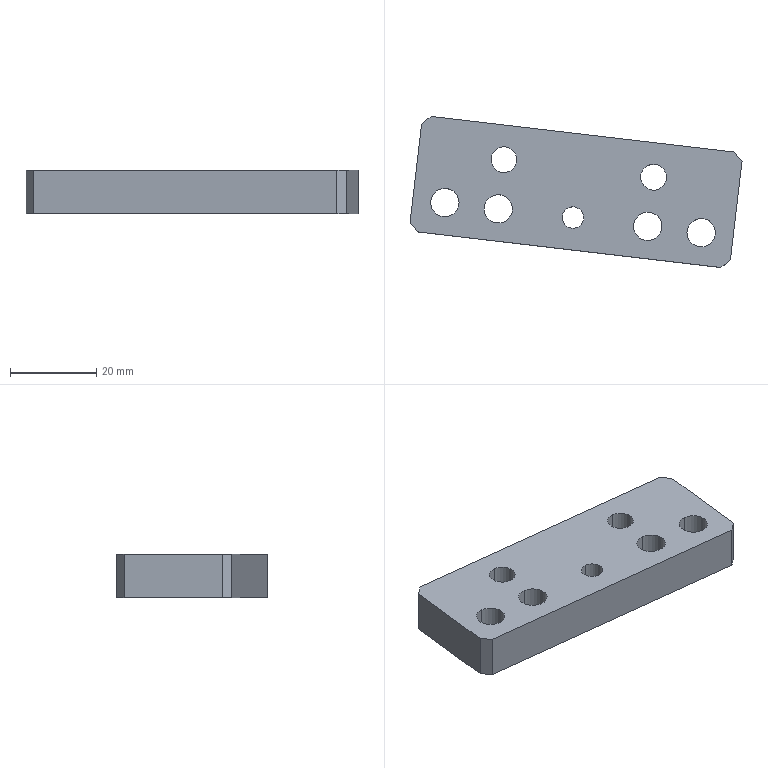Component | SolidWorks | 8TC-A17001-90-06EdgePressingRollerLockPlate-1 | 1 solid | 24 faces | box 77.17 x 35.1 x 10 mm | volume 18040 mm3 | cylinder 14 | plane 10 | commonest cylinder face diameters 6.6 x8 6 x4 5 x2 | material A3
build123d program:
from build123d import *

# Parameters (mm, degrees)
SKETCH1_W                     = 27
SKETCH1_H                     = 75
BOSS_EXTRUDE1_DEPTH           = 10
CHAMFER1_SIZE                 = 2
M6_CLEARANCE_HOLE_1_D         = 6.6
SIZE_MM_DOWEL_PIN_HOLE2_D     = 6
SIZE_MM_DOWEL_PIN_HOLE2_DEPTH = 10
SIZE_MM_DOWEL_PIN_HOLE2_TIP   = 1.803
M6_TAPPED_HOLE1_D             = 5


with BuildPart() as part:
    # Sketch1 → Boss-Extrude1 (new body)
    with BuildSketch(Plane.XY):
        Rectangle(SKETCH1_W, SKETCH1_H)
    extrude(amount=BOSS_EXTRUDE1_DEPTH)

    # Chamfer1
    chamfer1_edges = [part.edges().sort_by_distance(p)[0] for p in [
        (-13.5, 37.5, 5),
        (13.5, 37.5, 5),
        (13.5, -37.5, 5),
        (-13.5, -37.5, 5),
    ]]
    chamfer(chamfer1_edges, length=CHAMFER1_SIZE)

    # M6 Clearance Hole 1 (through all)
    with Locations(Plane.XY.offset(10)):
        with Locations((-6, 30), (-6, -30), (-6, 17.5), (-6, -17.5)):
            Hole(M6_CLEARANCE_HOLE_1_D / 2)

    # Size mm Dowel Pin Hole2
    with Locations(Plane.XY.offset(10)):
        with Locations((5.5, 17.5), (5.5, -17.5)):
            Hole(SIZE_MM_DOWEL_PIN_HOLE2_D / 2, depth=SIZE_MM_DOWEL_PIN_HOLE2_DEPTH)
            with Locations((0, 0, -(SIZE_MM_DOWEL_PIN_HOLE2_DEPTH + SIZE_MM_DOWEL_PIN_HOLE2_TIP / 2))):  # 118° drill point
                Cone(0, SIZE_MM_DOWEL_PIN_HOLE2_D / 2, SIZE_MM_DOWEL_PIN_HOLE2_TIP, mode=Mode.SUBTRACT)

    # M6 Tapped Hole1 (through all)
    with Locations(Plane.XY.offset(10)):
        with Locations((-6, 0)):
            Hole(M6_TAPPED_HOLE1_D / 2)


solid = part.part

# Placed as in the assembly
solid = solid.moved(Location((0.4951, -88.041, -136.2), (-180, 0, -83.3)))
STEP:
#1=CARTESIAN_POINT('',(-0.01955,-3.799,-5.362));
#2=VERTEX_POINT('',#1);
#3=CARTESIAN_POINT('',(0.003417,-3.603,-5.362));
#4=VERTEX_POINT('',#3);
#5=CARTESIAN_POINT('',(-0.008066,-3.701,-5.362));
#6=DIRECTION('',(-0.,0.,-1.));
#7=DIRECTION('',(0.1167,0.9932,0.));
#8=AXIS2_PLACEMENT_3D('',#5,#6,#7);
#9=CIRCLE('',#8,0.09843);
#10=EDGE_CURVE('',#2,#4,#9,.T.);
#11=ORIENTED_EDGE('',*,*,#10,.F.);
#12=CARTESIAN_POINT('',(-0.01955,-3.799,-5.756));
#13=VERTEX_POINT('',#12);
#14=CARTESIAN_POINT('',(-0.01955,-3.799,-5.756));
#15=DIRECTION('',(-0.,0.,-1.));
#16=VECTOR('',#15,39.37);
#17=LINE('',#14,#16);
#18=EDGE_CURVE('',#2,#13,#17,.T.);
#19=ORIENTED_EDGE('',*,*,#18,.T.);
#20=CARTESIAN_POINT('',(0.003417,-3.603,-5.756));
#21=VERTEX_POINT('',#20);
#22=CARTESIAN_POINT('',(-0.008066,-3.701,-5.756));
#23=DIRECTION('',(-0.,0.,-1.));
#24=DIRECTION('',(0.1167,0.9932,0.));
#25=AXIS2_PLACEMENT_3D('',#22,#23,#24);
#26=CIRCLE('',#25,0.09843);
#27=EDGE_CURVE('',#13,#21,#26,.T.);
#28=ORIENTED_EDGE('',*,*,#27,.T.);
#29=CARTESIAN_POINT('',(0.003417,-3.603,-5.756));
#30=DIRECTION('',(-0.,0.,-1.));
#31=VECTOR('',#30,39.37);
#32=LINE('',#29,#31);
#33=EDGE_CURVE('',#4,#21,#32,.T.);
#34=ORIENTED_EDGE('',*,*,#33,.F.);
#35=EDGE_LOOP('',(#11,#19,#28,#34));
#36=FACE_OUTER_BOUND('',#35,.T.);
#37=CARTESIAN_POINT('',(-0.008066,-3.701,-5.756));
#38=DIRECTION('',(-0.,0.,-1.));
#39=DIRECTION('',(0.1167,0.9932,0.));
#40=AXIS2_PLACEMENT_3D('',#37,#38,#39);
#41=CYLINDRICAL_SURFACE('',#40,0.09843);
#42=ADVANCED_FACE('',(#36),#41,.F.);
#43=CARTESIAN_POINT('',(0.7152,-3.449,-5.362));
#44=VERTEX_POINT('',#43);
#45=CARTESIAN_POINT('',(0.7428,-3.214,-5.362));
#46=VERTEX_POINT('',#45);
#47=CARTESIAN_POINT('',(0.729,-3.332,-5.362));
#48=DIRECTION('',(-0.,0.,-1.));
#49=DIRECTION('',(0.1167,0.9932,0.));
#50=AXIS2_PLACEMENT_3D('',#47,#48,#49);
#51=CIRCLE('',#50,0.1181);
#52=EDGE_CURVE('',#44,#46,#51,.T.);
#53=ORIENTED_EDGE('',*,*,#52,.F.);
#54=CARTESIAN_POINT('',(0.7152,-3.449,-5.756));
#55=VERTEX_POINT('',#54);
#56=CARTESIAN_POINT('',(0.7152,-3.449,-5.756));
#57=DIRECTION('',(-0.,0.,-1.));
#58=VECTOR('',#57,39.37);
#59=LINE('',#56,#58);
#60=EDGE_CURVE('',#44,#55,#59,.T.);
#61=ORIENTED_EDGE('',*,*,#60,.T.);
#62=CARTESIAN_POINT('',(0.7428,-3.214,-5.756));
#63=VERTEX_POINT('',#62);
#64=CARTESIAN_POINT('',(0.729,-3.332,-5.756));
#65=DIRECTION('',(-0.,0.,-1.));
#66=DIRECTION('',(0.1167,0.9932,0.));
#67=AXIS2_PLACEMENT_3D('',#64,#65,#66);
#68=CIRCLE('',#67,0.1181);
#69=EDGE_CURVE('',#55,#63,#68,.T.);
#70=ORIENTED_EDGE('',*,*,#69,.T.);
#71=CARTESIAN_POINT('',(0.7428,-3.214,-5.756));
#72=DIRECTION('',(-0.,0.,-1.));
#73=VECTOR('',#72,39.37);
#74=LINE('',#71,#73);
#75=EDGE_CURVE('',#46,#63,#74,.T.);
#76=ORIENTED_EDGE('',*,*,#75,.F.);
#77=EDGE_LOOP('',(#53,#61,#70,#76));
#78=FACE_OUTER_BOUND('',#77,.T.);
#79=CARTESIAN_POINT('',(0.729,-3.332,-5.756));
#80=DIRECTION('',(-0.,0.,-1.));
#81=DIRECTION('',(0.1167,0.9932,0.));
#82=AXIS2_PLACEMENT_3D('',#79,#80,#81);
#83=CYLINDRICAL_SURFACE('',#82,0.1181);
#84=ADVANCED_FACE('',(#78),#83,.F.);
#85=CARTESIAN_POINT('',(-0.6533,-3.288,-5.362));
#86=VERTEX_POINT('',#85);
#87=CARTESIAN_POINT('',(-0.6257,-3.053,-5.362));
#88=VERTEX_POINT('',#87);
#89=CARTESIAN_POINT('',(-0.6395,-3.171,-5.362));
#90=DIRECTION('',(-0.,0.,-1.));
#91=DIRECTION('',(0.1167,0.9932,0.));
#92=AXIS2_PLACEMENT_3D('',#89,#90,#91);
#93=CIRCLE('',#92,0.1181);
#94=EDGE_CURVE('',#86,#88,#93,.T.);
#95=ORIENTED_EDGE('',*,*,#94,.F.);
#96=CARTESIAN_POINT('',(-0.6533,-3.288,-5.756));
#97=VERTEX_POINT('',#96);
#98=CARTESIAN_POINT('',(-0.6533,-3.288,-5.756));
#99=DIRECTION('',(-0.,0.,-1.));
#100=VECTOR('',#99,39.37);
#101=LINE('',#98,#100);
#102=EDGE_CURVE('',#86,#97,#101,.T.);
#103=ORIENTED_EDGE('',*,*,#102,.T.);
#104=CARTESIAN_POINT('',(-0.6257,-3.053,-5.756));
#105=VERTEX_POINT('',#104);
#106=CARTESIAN_POINT('',(-0.6395,-3.171,-5.756));
#107=DIRECTION('',(-0.,0.,-1.));
#108=DIRECTION('',(0.1167,0.9932,0.));
#109=AXIS2_PLACEMENT_3D('',#106,#107,#108);
#110=CIRCLE('',#109,0.1181);
#111=EDGE_CURVE('',#97,#105,#110,.T.);
#112=ORIENTED_EDGE('',*,*,#111,.T.);
#113=CARTESIAN_POINT('',(-0.6257,-3.053,-5.756));
#114=DIRECTION('',(-0.,0.,-1.));
#115=VECTOR('',#114,39.37);
#116=LINE('',#113,#115);
#117=EDGE_CURVE('',#88,#105,#116,.T.);
#118=ORIENTED_EDGE('',*,*,#117,.F.);
#119=EDGE_LOOP('',(#95,#103,#112,#118));
#120=FACE_OUTER_BOUND('',#119,.T.);
#121=CARTESIAN_POINT('',(-0.6395,-3.171,-5.756));
#122=DIRECTION('',(-0.,0.,-1.));
#123=DIRECTION('',(0.1167,0.9932,0.));
#124=AXIS2_PLACEMENT_3D('',#121,#122,#123);
#125=CYLINDRICAL_SURFACE('',#124,0.1181);
#126=ADVANCED_FACE('',(#120),#125,.F.);
#127=CARTESIAN_POINT('',(1.15,-3.968,-5.362));
#128=VERTEX_POINT('',#127);
#129=CARTESIAN_POINT('',(1.18,-3.71,-5.362));
#130=VERTEX_POINT('',#129);
#131=CARTESIAN_POINT('',(1.165,-3.839,-5.362));
#132=DIRECTION('',(-0.,0.,-1.));
#133=DIRECTION('',(0.1167,0.9932,0.));
#134=AXIS2_PLACEMENT_3D('',#131,#132,#133);
#135=CIRCLE('',#134,0.1299);
#136=EDGE_CURVE('',#128,#130,#135,.T.);
#137=ORIENTED_EDGE('',*,*,#136,.F.);
#138=CARTESIAN_POINT('',(1.15,-3.968,-5.756));
#139=VERTEX_POINT('',#138);
#140=CARTESIAN_POINT('',(1.15,-3.968,-5.756));
#141=DIRECTION('',(-0.,0.,-1.));
#142=VECTOR('',#141,39.37);
#143=LINE('',#140,#142);
#144=EDGE_CURVE('',#128,#139,#143,.T.);
#145=ORIENTED_EDGE('',*,*,#144,.T.);
#146=CARTESIAN_POINT('',(1.18,-3.71,-5.756));
#147=VERTEX_POINT('',#146);
#148=CARTESIAN_POINT('',(1.165,-3.839,-5.756));
#149=DIRECTION('',(-0.,0.,-1.));
#150=DIRECTION('',(0.1167,0.9932,0.));
#151=AXIS2_PLACEMENT_3D('',#148,#149,#150);
#152=CIRCLE('',#151,0.1299);
#153=EDGE_CURVE('',#139,#147,#152,.T.);
#154=ORIENTED_EDGE('',*,*,#153,.T.);
#155=CARTESIAN_POINT('',(1.18,-3.71,-5.756));
#156=DIRECTION('',(-0.,0.,-1.));
#157=VECTOR('',#156,39.37);
#158=LINE('',#155,#157);
#159=EDGE_CURVE('',#130,#147,#158,.T.);
#160=ORIENTED_EDGE('',*,*,#159,.F.);
#161=EDGE_LOOP('',(#137,#145,#154,#160));
#162=FACE_OUTER_BOUND('',#161,.T.);
#163=CARTESIAN_POINT('',(1.165,-3.839,-5.756));
#164=DIRECTION('',(-0.,0.,-1.));
#165=DIRECTION('',(0.1167,0.9932,0.));
#166=AXIS2_PLACEMENT_3D('',#163,#164,#165);
#167=CYLINDRICAL_SURFACE('',#166,0.1299);
#168=ADVANCED_FACE('',(#162),#167,.F.);
#169=CARTESIAN_POINT('',(-1.196,-3.692,-5.362));
#170=VERTEX_POINT('',#169);
#171=CARTESIAN_POINT('',(-1.166,-3.434,-5.362));
#172=VERTEX_POINT('',#171);
#173=CARTESIAN_POINT('',(-1.181,-3.563,-5.362));
#174=DIRECTION('',(-0.,0.,-1.));
#175=DIRECTION('',(0.1167,0.9932,0.));
#176=AXIS2_PLACEMENT_3D('',#173,#174,#175);
#177=CIRCLE('',#176,0.1299);
#178=EDGE_CURVE('',#170,#172,#177,.T.);
#179=ORIENTED_EDGE('',*,*,#178,.F.);
#180=CARTESIAN_POINT('',(-1.196,-3.692,-5.756));
#181=VERTEX_POINT('',#180);
#182=CARTESIAN_POINT('',(-1.196,-3.692,-5.756));
#183=DIRECTION('',(-0.,0.,-1.));
#184=VECTOR('',#183,39.37);
#185=LINE('',#182,#184);
#186=EDGE_CURVE('',#170,#181,#185,.T.);
#187=ORIENTED_EDGE('',*,*,#186,.T.);
#188=CARTESIAN_POINT('',(-1.166,-3.434,-5.756));
#189=VERTEX_POINT('',#188);
#190=CARTESIAN_POINT('',(-1.181,-3.563,-5.756));
#191=DIRECTION('',(-0.,0.,-1.));
#192=DIRECTION('',(0.1167,0.9932,0.));
#193=AXIS2_PLACEMENT_3D('',#190,#191,#192);
#194=CIRCLE('',#193,0.1299);
#195=EDGE_CURVE('',#181,#189,#194,.T.);
#196=ORIENTED_EDGE('',*,*,#195,.T.);
#197=CARTESIAN_POINT('',(-1.166,-3.434,-5.756));
#198=DIRECTION('',(-0.,0.,-1.));
#199=VECTOR('',#198,39.37);
#200=LINE('',#197,#199);
#201=EDGE_CURVE('',#172,#189,#200,.T.);
#202=ORIENTED_EDGE('',*,*,#201,.F.);
#203=EDGE_LOOP('',(#179,#187,#196,#202));
#204=FACE_OUTER_BOUND('',#203,.T.);
#205=CARTESIAN_POINT('',(-1.181,-3.563,-5.756));
#206=DIRECTION('',(-0.,0.,-1.));
#207=DIRECTION('',(0.1167,0.9932,0.));
#208=AXIS2_PLACEMENT_3D('',#205,#206,#207);
#209=CYLINDRICAL_SURFACE('',#208,0.1299);
#210=ADVANCED_FACE('',(#204),#209,.F.);
#211=CARTESIAN_POINT('',(0.661,-3.91,-5.362));
#212=VERTEX_POINT('',#211);
#213=CARTESIAN_POINT('',(0.6914,-3.652,-5.362));
#214=VERTEX_POINT('',#213);
#215=CARTESIAN_POINT('',(0.6762,-3.781,-5.362));
#216=DIRECTION('',(-0.,0.,-1.));
#217=DIRECTION('',(0.1167,0.9932,0.));
#218=AXIS2_PLACEMENT_3D('',#215,#216,#217);
#219=CIRCLE('',#218,0.1299);
#220=EDGE_CURVE('',#212,#214,#219,.T.);
#221=ORIENTED_EDGE('',*,*,#220,.F.);
#222=CARTESIAN_POINT('',(0.661,-3.91,-5.756));
#223=VERTEX_POINT('',#222);
#224=CARTESIAN_POINT('',(0.661,-3.91,-5.756));
#225=DIRECTION('',(-0.,0.,-1.));
#226=VECTOR('',#225,39.37);
#227=LINE('',#224,#226);
#228=EDGE_CURVE('',#212,#223,#227,.T.);
#229=ORIENTED_EDGE('',*,*,#228,.T.);
#230=CARTESIAN_POINT('',(0.6914,-3.652,-5.756));
#231=VERTEX_POINT('',#230);
#232=CARTESIAN_POINT('',(0.6762,-3.781,-5.756));
#233=DIRECTION('',(-0.,0.,-1.));
#234=DIRECTION('',(0.1167,0.9932,0.));
#235=AXIS2_PLACEMENT_3D('',#232,#233,#234);
#236=CIRCLE('',#235,0.1299);
#237=EDGE_CURVE('',#223,#231,#236,.T.);
#238=ORIENTED_EDGE('',*,*,#237,.T.);
#239=CARTESIAN_POINT('',(0.6914,-3.652,-5.756));
#240=DIRECTION('',(-0.,0.,-1.));
#241=VECTOR('',#240,39.37);
#242=LINE('',#239,#241);
#243=EDGE_CURVE('',#214,#231,#242,.T.);
#244=ORIENTED_EDGE('',*,*,#243,.F.);
#245=EDGE_LOOP('',(#221,#229,#238,#244));
#246=FACE_OUTER_BOUND('',#245,.T.);
#247=CARTESIAN_POINT('',(0.6762,-3.781,-5.756));
#248=DIRECTION('',(-0.,0.,-1.));
#249=DIRECTION('',(0.1167,0.9932,0.));
#250=AXIS2_PLACEMENT_3D('',#247,#248,#249);
#251=CYLINDRICAL_SURFACE('',#250,0.1299);
#252=ADVANCED_FACE('',(#246),#251,.F.);
#253=CARTESIAN_POINT('',(-0.7075,-3.749,-5.362));
#254=VERTEX_POINT('',#253);
#255=CARTESIAN_POINT('',(-0.6772,-3.491,-5.362));
#256=VERTEX_POINT('',#255);
#257=CARTESIAN_POINT('',(-0.6923,-3.62,-5.362));
#258=DIRECTION('',(-0.,0.,-1.));
#259=DIRECTION('',(0.1167,0.9932,0.));
#260=AXIS2_PLACEMENT_3D('',#257,#258,#259);
#261=CIRCLE('',#260,0.1299);
#262=EDGE_CURVE('',#254,#256,#261,.T.);
#263=ORIENTED_EDGE('',*,*,#262,.F.);
#264=CARTESIAN_POINT('',(-0.7075,-3.749,-5.756));
#265=VERTEX_POINT('',#264);
#266=CARTESIAN_POINT('',(-0.7075,-3.749,-5.756));
#267=DIRECTION('',(-0.,0.,-1.));
#268=VECTOR('',#267,39.37);
#269=LINE('',#266,#268);
#270=EDGE_CURVE('',#254,#265,#269,.T.);
#271=ORIENTED_EDGE('',*,*,#270,.T.);
#272=CARTESIAN_POINT('',(-0.6772,-3.491,-5.756));
#273=VERTEX_POINT('',#272);
#274=CARTESIAN_POINT('',(-0.6923,-3.62,-5.756));
#275=DIRECTION('',(-0.,0.,-1.));
#276=DIRECTION('',(0.1167,0.9932,0.));
#277=AXIS2_PLACEMENT_3D('',#274,#275,#276);
#278=CIRCLE('',#277,0.1299);
#279=EDGE_CURVE('',#265,#273,#278,.T.);
#280=ORIENTED_EDGE('',*,*,#279,.T.);
#281=CARTESIAN_POINT('',(-0.6772,-3.491,-5.756));
#282=DIRECTION('',(-0.,0.,-1.));
#283=VECTOR('',#282,39.37);
#284=LINE('',#281,#283);
#285=EDGE_CURVE('',#256,#273,#284,.T.);
#286=ORIENTED_EDGE('',*,*,#285,.F.);
#287=EDGE_LOOP('',(#263,#271,#280,#286));
#288=FACE_OUTER_BOUND('',#287,.T.);
#289=CARTESIAN_POINT('',(-0.6923,-3.62,-5.756));
#290=DIRECTION('',(-0.,0.,-1.));
#291=DIRECTION('',(0.1167,0.9932,0.));
#292=AXIS2_PLACEMENT_3D('',#289,#290,#291);
#293=CYLINDRICAL_SURFACE('',#292,0.1299);
#294=ADVANCED_FACE('',(#288),#293,.F.);
#295=CARTESIAN_POINT('',(1.346,-4.157,-5.362));
#296=VERTEX_POINT('',#295);
#297=CARTESIAN_POINT('',(-1.431,-3.831,-5.362));
#298=VERTEX_POINT('',#297);
#299=CARTESIAN_POINT('',(1.424,-4.166,-5.362));
#300=DIRECTION('',(-0.9932,0.1167,0.));
#301=VECTOR('',#300,39.37);
#302=LINE('',#299,#301);
#303=EDGE_CURVE('',#296,#298,#302,.T.);
#304=ORIENTED_EDGE('',*,*,#303,.T.);
#305=CARTESIAN_POINT('',(-1.431,-3.831,-5.756));
#306=VERTEX_POINT('',#305);
#307=CARTESIAN_POINT('',(-1.431,-3.831,-5.756));
#308=DIRECTION('',(-0.,0.,-1.));
#309=VECTOR('',#308,39.37);
#310=LINE('',#307,#309);
#311=EDGE_CURVE('',#298,#306,#310,.T.);
#312=ORIENTED_EDGE('',*,*,#311,.T.);
#313=CARTESIAN_POINT('',(1.346,-4.157,-5.756));
#314=VERTEX_POINT('',#313);
#315=CARTESIAN_POINT('',(1.424,-4.166,-5.756));
#316=DIRECTION('',(-0.9932,0.1167,0.));
#317=VECTOR('',#316,39.37);
#318=LINE('',#315,#317);
#319=EDGE_CURVE('',#314,#306,#318,.T.);
#320=ORIENTED_EDGE('',*,*,#319,.F.);
#321=CARTESIAN_POINT('',(1.346,-4.157,-5.756));
#322=DIRECTION('',(0.,-0.,1.));
#323=VECTOR('',#322,39.37);
#324=LINE('',#321,#323);
#325=EDGE_CURVE('',#314,#296,#324,.T.);
#326=ORIENTED_EDGE('',*,*,#325,.T.);
#327=EDGE_LOOP('',(#304,#312,#320,#326));
#328=FACE_OUTER_BOUND('',#327,.T.);
#329=CARTESIAN_POINT('',(1.424,-4.166,-5.756));
#330=DIRECTION('',(0.1167,0.9932,0.));
#331=DIRECTION('',(0.9932,-0.1167,-0.));
#332=AXIS2_PLACEMENT_3D('',#329,#330,#331);
#333=PLANE('',#332);
#334=ADVANCED_FACE('',(#328),#333,.F.);
#335=CARTESIAN_POINT('',(-1.5,-3.744,-5.756));
#336=VERTEX_POINT('',#335);
#337=CARTESIAN_POINT('',(-1.394,-2.844,-5.756));
#338=VERTEX_POINT('',#337);
#339=CARTESIAN_POINT('',(-1.385,-2.766,-5.756));
#340=DIRECTION('',(0.1167,0.9932,0.));
#341=VECTOR('',#340,39.37);
#342=LINE('',#339,#341);
#343=EDGE_CURVE('',#336,#338,#342,.T.);
#344=ORIENTED_EDGE('',*,*,#343,.F.);
#345=CARTESIAN_POINT('',(-1.5,-3.744,-5.362));
#346=VERTEX_POINT('',#345);
#347=CARTESIAN_POINT('',(-1.5,-3.744,-5.756));
#348=DIRECTION('',(0.,-0.,1.));
#349=VECTOR('',#348,39.37);
#350=LINE('',#347,#349);
#351=EDGE_CURVE('',#336,#346,#350,.T.);
#352=ORIENTED_EDGE('',*,*,#351,.T.);
#353=CARTESIAN_POINT('',(-1.394,-2.844,-5.362));
#354=VERTEX_POINT('',#353);
#355=CARTESIAN_POINT('',(-1.385,-2.766,-5.362));
#356=DIRECTION('',(0.1167,0.9932,0.));
#357=VECTOR('',#356,39.37);
#358=LINE('',#355,#357);
#359=EDGE_CURVE('',#346,#354,#358,.T.);
#360=ORIENTED_EDGE('',*,*,#359,.T.);
#361=CARTESIAN_POINT('',(-1.394,-2.844,-5.756));
#362=DIRECTION('',(-0.,0.,-1.));
#363=VECTOR('',#362,39.37);
#364=LINE('',#361,#363);
#365=EDGE_CURVE('',#354,#338,#364,.T.);
#366=ORIENTED_EDGE('',*,*,#365,.T.);
#367=EDGE_LOOP('',(#344,#352,#360,#366));
#368=FACE_OUTER_BOUND('',#367,.T.);
#369=CARTESIAN_POINT('',(-1.385,-2.766,-5.756));
#370=DIRECTION('',(0.9932,-0.1167,-0.));
#371=DIRECTION('',(-0.,0.,-1.));
#372=AXIS2_PLACEMENT_3D('',#369,#370,#371);
#373=PLANE('',#372);
#374=ADVANCED_FACE('',(#368),#373,.F.);
#375=CARTESIAN_POINT('',(-1.307,-2.775,-5.756));
#376=VERTEX_POINT('',#375);
#377=CARTESIAN_POINT('',(1.47,-3.101,-5.756));
#378=VERTEX_POINT('',#377);
#379=CARTESIAN_POINT('',(1.548,-3.111,-5.756));
#380=DIRECTION('',(0.9932,-0.1167,-0.));
#381=VECTOR('',#380,39.37);
#382=LINE('',#379,#381);
#383=EDGE_CURVE('',#376,#378,#382,.T.);
#384=ORIENTED_EDGE('',*,*,#383,.F.);
#385=CARTESIAN_POINT('',(-1.307,-2.775,-5.362));
#386=VERTEX_POINT('',#385);
#387=CARTESIAN_POINT('',(-1.307,-2.775,-5.756));
#388=DIRECTION('',(0.,-0.,1.));
#389=VECTOR('',#388,39.37);
#390=LINE('',#387,#389);
#391=EDGE_CURVE('',#376,#386,#390,.T.);
#392=ORIENTED_EDGE('',*,*,#391,.T.);
#393=CARTESIAN_POINT('',(1.47,-3.101,-5.362));
#394=VERTEX_POINT('',#393);
#395=CARTESIAN_POINT('',(1.548,-3.111,-5.362));
#396=DIRECTION('',(0.9932,-0.1167,-0.));
#397=VECTOR('',#396,39.37);
#398=LINE('',#395,#397);
#399=EDGE_CURVE('',#386,#394,#398,.T.);
#400=ORIENTED_EDGE('',*,*,#399,.T.);
#401=CARTESIAN_POINT('',(1.47,-3.101,-5.756));
#402=DIRECTION('',(-0.,0.,-1.));
#403=VECTOR('',#402,39.37);
#404=LINE('',#401,#403);
#405=EDGE_CURVE('',#394,#378,#404,.T.);
#406=ORIENTED_EDGE('',*,*,#405,.T.);
#407=EDGE_LOOP('',(#384,#392,#400,#406));
#408=FACE_OUTER_BOUND('',#407,.T.);
#409=CARTESIAN_POINT('',(1.548,-3.111,-5.756));
#410=DIRECTION('',(-0.1167,-0.9932,-0.));
#411=DIRECTION('',(-0.9932,0.1167,0.));
#412=AXIS2_PLACEMENT_3D('',#409,#410,#411);
#413=PLANE('',#412);
#414=ADVANCED_FACE('',(#408),#413,.F.);
#415=CARTESIAN_POINT('',(1.539,-3.189,-5.362));
#416=VERTEX_POINT('',#415);
#417=CARTESIAN_POINT('',(1.433,-4.088,-5.362));
#418=VERTEX_POINT('',#417);
#419=CARTESIAN_POINT('',(1.548,-3.111,-5.362));
#420=DIRECTION('',(-0.1167,-0.9932,-0.));
#421=VECTOR('',#420,39.37);
#422=LINE('',#419,#421);
#423=EDGE_CURVE('',#416,#418,#422,.T.);
#424=ORIENTED_EDGE('',*,*,#423,.T.);
#425=CARTESIAN_POINT('',(1.433,-4.088,-5.756));
#426=VERTEX_POINT('',#425);
#427=CARTESIAN_POINT('',(1.433,-4.088,-5.756));
#428=DIRECTION('',(-0.,0.,-1.));
#429=VECTOR('',#428,39.37);
#430=LINE('',#427,#429);
#431=EDGE_CURVE('',#418,#426,#430,.T.);
#432=ORIENTED_EDGE('',*,*,#431,.T.);
#433=CARTESIAN_POINT('',(1.539,-3.189,-5.756));
#434=VERTEX_POINT('',#433);
#435=CARTESIAN_POINT('',(1.548,-3.111,-5.756));
#436=DIRECTION('',(-0.1167,-0.9932,-0.));
#437=VECTOR('',#436,39.37);
#438=LINE('',#435,#437);
#439=EDGE_CURVE('',#434,#426,#438,.T.);
#440=ORIENTED_EDGE('',*,*,#439,.F.);
#441=CARTESIAN_POINT('',(1.539,-3.189,-5.756));
#442=DIRECTION('',(0.,-0.,1.));
#443=VECTOR('',#442,39.37);
#444=LINE('',#441,#443);
#445=EDGE_CURVE('',#434,#416,#444,.T.);
#446=ORIENTED_EDGE('',*,*,#445,.T.);
#447=EDGE_LOOP('',(#424,#432,#440,#446));
#448=FACE_OUTER_BOUND('',#447,.T.);
#449=CARTESIAN_POINT('',(1.548,-3.111,-5.756));
#450=DIRECTION('',(-0.9932,0.1167,0.));
#451=DIRECTION('',(0.,-0.,1.));
#452=AXIS2_PLACEMENT_3D('',#449,#450,#451);
#453=PLANE('',#452);
#454=ADVANCED_FACE('',(#448),#453,.F.);
#455=CARTESIAN_POINT('',(-0.008066,-3.701,-5.756));
#456=DIRECTION('',(-0.,0.,-1.));
#457=DIRECTION('',(0.1167,0.9932,0.));
#458=AXIS2_PLACEMENT_3D('',#455,#456,#457);
#459=CIRCLE('',#458,0.09843);
#460=EDGE_CURVE('',#21,#13,#459,.T.);
#461=ORIENTED_EDGE('',*,*,#460,.F.);
#462=ORIENTED_EDGE('',*,*,#27,.F.);
#463=EDGE_LOOP('',(#461,#462));
#464=FACE_BOUND('',#463,.T.);
#465=CARTESIAN_POINT('',(0.729,-3.332,-5.756));
#466=DIRECTION('',(-0.,0.,-1.));
#467=DIRECTION('',(0.1167,0.9932,0.));
#468=AXIS2_PLACEMENT_3D('',#465,#466,#467);
#469=CIRCLE('',#468,0.1181);
#470=EDGE_CURVE('',#63,#55,#469,.T.);
#471=ORIENTED_EDGE('',*,*,#470,.F.);
#472=ORIENTED_EDGE('',*,*,#69,.F.);
#473=EDGE_LOOP('',(#471,#472));
#474=FACE_BOUND('',#473,.T.);
#475=CARTESIAN_POINT('',(-0.6395,-3.171,-5.756));
#476=DIRECTION('',(-0.,0.,-1.));
#477=DIRECTION('',(0.1167,0.9932,0.));
#478=AXIS2_PLACEMENT_3D('',#475,#476,#477);
#479=CIRCLE('',#478,0.1181);
#480=EDGE_CURVE('',#105,#97,#479,.T.);
#481=ORIENTED_EDGE('',*,*,#480,.F.);
#482=ORIENTED_EDGE('',*,*,#111,.F.);
#483=EDGE_LOOP('',(#481,#482));
#484=FACE_BOUND('',#483,.T.);
#485=CARTESIAN_POINT('',(1.165,-3.839,-5.756));
#486=DIRECTION('',(-0.,0.,-1.));
#487=DIRECTION('',(0.1167,0.9932,0.));
#488=AXIS2_PLACEMENT_3D('',#485,#486,#487);
#489=CIRCLE('',#488,0.1299);
#490=EDGE_CURVE('',#147,#139,#489,.T.);
#491=ORIENTED_EDGE('',*,*,#490,.F.);
#492=ORIENTED_EDGE('',*,*,#153,.F.);
#493=EDGE_LOOP('',(#491,#492));
#494=FACE_BOUND('',#493,.T.);
#495=CARTESIAN_POINT('',(-1.181,-3.563,-5.756));
#496=DIRECTION('',(-0.,0.,-1.));
#497=DIRECTION('',(0.1167,0.9932,0.));
#498=AXIS2_PLACEMENT_3D('',#495,#496,#497);
#499=CIRCLE('',#498,0.1299);
#500=EDGE_CURVE('',#189,#181,#499,.T.);
#501=ORIENTED_EDGE('',*,*,#500,.F.);
#502=ORIENTED_EDGE('',*,*,#195,.F.);
#503=EDGE_LOOP('',(#501,#502));
#504=FACE_BOUND('',#503,.T.);
#505=CARTESIAN_POINT('',(0.6762,-3.781,-5.756));
#506=DIRECTION('',(-0.,0.,-1.));
#507=DIRECTION('',(0.1167,0.9932,0.));
#508=AXIS2_PLACEMENT_3D('',#505,#506,#507);
#509=CIRCLE('',#508,0.1299);
#510=EDGE_CURVE('',#231,#223,#509,.T.);
#511=ORIENTED_EDGE('',*,*,#510,.F.);
#512=ORIENTED_EDGE('',*,*,#237,.F.);
#513=EDGE_LOOP('',(#511,#512));
#514=FACE_BOUND('',#513,.T.);
#515=CARTESIAN_POINT('',(-0.6923,-3.62,-5.756));
#516=DIRECTION('',(-0.,0.,-1.));
#517=DIRECTION('',(0.1167,0.9932,0.));
#518=AXIS2_PLACEMENT_3D('',#515,#516,#517);
#519=CIRCLE('',#518,0.1299);
#520=EDGE_CURVE('',#273,#265,#519,.T.);
#521=ORIENTED_EDGE('',*,*,#520,.F.);
#522=ORIENTED_EDGE('',*,*,#279,.F.);
#523=EDGE_LOOP('',(#521,#522));
#524=FACE_BOUND('',#523,.T.);
#525=ORIENTED_EDGE('',*,*,#319,.T.);
#526=CARTESIAN_POINT('',(-1.5,-3.744,-5.756));
#527=DIRECTION('',(-0.6198,0.7848,0.));
#528=VECTOR('',#527,39.37);
#529=LINE('',#526,#528);
#530=EDGE_CURVE('',#306,#336,#529,.T.);
#531=ORIENTED_EDGE('',*,*,#530,.T.);
#532=ORIENTED_EDGE('',*,*,#343,.T.);
#533=CARTESIAN_POINT('',(-1.307,-2.775,-5.756));
#534=DIRECTION('',(0.7848,0.6198,0.));
#535=VECTOR('',#534,39.37);
#536=LINE('',#533,#535);
#537=EDGE_CURVE('',#338,#376,#536,.T.);
#538=ORIENTED_EDGE('',*,*,#537,.T.);
#539=ORIENTED_EDGE('',*,*,#383,.T.);
#540=CARTESIAN_POINT('',(1.539,-3.189,-5.756));
#541=DIRECTION('',(0.6198,-0.7848,-0.));
#542=VECTOR('',#541,39.37);
#543=LINE('',#540,#542);
#544=EDGE_CURVE('',#378,#434,#543,.T.);
#545=ORIENTED_EDGE('',*,*,#544,.T.);
#546=ORIENTED_EDGE('',*,*,#439,.T.);
#547=CARTESIAN_POINT('',(1.346,-4.157,-5.756));
#548=DIRECTION('',(-0.7848,-0.6198,-0.));
#549=VECTOR('',#548,39.37);
#550=LINE('',#547,#549);
#551=EDGE_CURVE('',#426,#314,#550,.T.);
#552=ORIENTED_EDGE('',*,*,#551,.T.);
#553=EDGE_LOOP('',(#525,#531,#532,#538,#539,#545,#546,#552));
#554=FACE_OUTER_BOUND('',#553,.T.);
#555=CARTESIAN_POINT('',(0.01949,-3.466,-5.756));
#556=DIRECTION('',(0.,-0.,1.));
#557=DIRECTION('',(-0.1167,-0.9932,-0.));
#558=AXIS2_PLACEMENT_3D('',#555,#556,#557);
#559=PLANE('',#558);
#560=ADVANCED_FACE('',(#464,#474,#484,#494,#504,#514,#524,#554),#559,.F.);
#561=CARTESIAN_POINT('',(-0.008066,-3.701,-5.362));
#562=DIRECTION('',(-0.,0.,-1.));
#563=DIRECTION('',(0.1167,0.9932,0.));
#564=AXIS2_PLACEMENT_3D('',#561,#562,#563);
#565=CIRCLE('',#564,0.09843);
#566=EDGE_CURVE('',#4,#2,#565,.T.);
#567=ORIENTED_EDGE('',*,*,#566,.T.);
#568=ORIENTED_EDGE('',*,*,#10,.T.);
#569=EDGE_LOOP('',(#567,#568));
#570=FACE_BOUND('',#569,.T.);
#571=CARTESIAN_POINT('',(0.729,-3.332,-5.362));
#572=DIRECTION('',(-0.,0.,-1.));
#573=DIRECTION('',(0.1167,0.9932,0.));
#574=AXIS2_PLACEMENT_3D('',#571,#572,#573);
#575=CIRCLE('',#574,0.1181);
#576=EDGE_CURVE('',#46,#44,#575,.T.);
#577=ORIENTED_EDGE('',*,*,#576,.T.);
#578=ORIENTED_EDGE('',*,*,#52,.T.);
#579=EDGE_LOOP('',(#577,#578));
#580=FACE_BOUND('',#579,.T.);
#581=CARTESIAN_POINT('',(-0.6395,-3.171,-5.362));
#582=DIRECTION('',(-0.,0.,-1.));
#583=DIRECTION('',(0.1167,0.9932,0.));
#584=AXIS2_PLACEMENT_3D('',#581,#582,#583);
#585=CIRCLE('',#584,0.1181);
#586=EDGE_CURVE('',#88,#86,#585,.T.);
#587=ORIENTED_EDGE('',*,*,#586,.T.);
#588=ORIENTED_EDGE('',*,*,#94,.T.);
#589=EDGE_LOOP('',(#587,#588));
#590=FACE_BOUND('',#589,.T.);
#591=CARTESIAN_POINT('',(1.165,-3.839,-5.362));
#592=DIRECTION('',(-0.,0.,-1.));
#593=DIRECTION('',(0.1167,0.9932,0.));
#594=AXIS2_PLACEMENT_3D('',#591,#592,#593);
#595=CIRCLE('',#594,0.1299);
#596=EDGE_CURVE('',#130,#128,#595,.T.);
#597=ORIENTED_EDGE('',*,*,#596,.T.);
#598=ORIENTED_EDGE('',*,*,#136,.T.);
#599=EDGE_LOOP('',(#597,#598));
#600=FACE_BOUND('',#599,.T.);
#601=CARTESIAN_POINT('',(-1.181,-3.563,-5.362));
#602=DIRECTION('',(-0.,0.,-1.));
#603=DIRECTION('',(0.1167,0.9932,0.));
#604=AXIS2_PLACEMENT_3D('',#601,#602,#603);
#605=CIRCLE('',#604,0.1299);
#606=EDGE_CURVE('',#172,#170,#605,.T.);
#607=ORIENTED_EDGE('',*,*,#606,.T.);
#608=ORIENTED_EDGE('',*,*,#178,.T.);
#609=EDGE_LOOP('',(#607,#608));
#610=FACE_BOUND('',#609,.T.);
#611=CARTESIAN_POINT('',(0.6762,-3.781,-5.362));
#612=DIRECTION('',(-0.,0.,-1.));
#613=DIRECTION('',(0.1167,0.9932,0.));
#614=AXIS2_PLACEMENT_3D('',#611,#612,#613);
#615=CIRCLE('',#614,0.1299);
#616=EDGE_CURVE('',#214,#212,#615,.T.);
#617=ORIENTED_EDGE('',*,*,#616,.T.);
#618=ORIENTED_EDGE('',*,*,#220,.T.);
#619=EDGE_LOOP('',(#617,#618));
#620=FACE_BOUND('',#619,.T.);
#621=CARTESIAN_POINT('',(-0.6923,-3.62,-5.362));
#622=DIRECTION('',(-0.,0.,-1.));
#623=DIRECTION('',(0.1167,0.9932,0.));
#624=AXIS2_PLACEMENT_3D('',#621,#622,#623);
#625=CIRCLE('',#624,0.1299);
#626=EDGE_CURVE('',#256,#254,#625,.T.);
#627=ORIENTED_EDGE('',*,*,#626,.T.);
#628=ORIENTED_EDGE('',*,*,#262,.T.);
#629=EDGE_LOOP('',(#627,#628));
#630=FACE_BOUND('',#629,.T.);
#631=ORIENTED_EDGE('',*,*,#359,.F.);
#632=CARTESIAN_POINT('',(-1.051,-4.312,-5.362));
#633=DIRECTION('',(0.6198,-0.7848,-0.));
#634=VECTOR('',#633,39.37);
#635=LINE('',#632,#634);
#636=EDGE_CURVE('',#346,#298,#635,.T.);
#637=ORIENTED_EDGE('',*,*,#636,.T.);
#638=ORIENTED_EDGE('',*,*,#303,.F.);
#639=CARTESIAN_POINT('',(0.8649,-4.537,-5.362));
#640=DIRECTION('',(0.7848,0.6198,0.));
#641=VECTOR('',#640,39.37);
#642=LINE('',#639,#641);
#643=EDGE_CURVE('',#296,#418,#642,.T.);
#644=ORIENTED_EDGE('',*,*,#643,.T.);
#645=ORIENTED_EDGE('',*,*,#423,.F.);
#646=CARTESIAN_POINT('',(1.09,-2.621,-5.362));
#647=DIRECTION('',(-0.6198,0.7848,0.));
#648=VECTOR('',#647,39.37);
#649=LINE('',#646,#648);
#650=EDGE_CURVE('',#416,#394,#649,.T.);
#651=ORIENTED_EDGE('',*,*,#650,.T.);
#652=ORIENTED_EDGE('',*,*,#399,.F.);
#653=CARTESIAN_POINT('',(-0.826,-2.396,-5.362));
#654=DIRECTION('',(-0.7848,-0.6198,-0.));
#655=VECTOR('',#654,39.37);
#656=LINE('',#653,#655);
#657=EDGE_CURVE('',#386,#354,#656,.T.);
#658=ORIENTED_EDGE('',*,*,#657,.T.);
#659=EDGE_LOOP('',(#631,#637,#638,#644,#645,#651,#652,#658));
#660=FACE_OUTER_BOUND('',#659,.T.);
#661=CARTESIAN_POINT('',(0.01949,-3.466,-5.362));
#662=DIRECTION('',(0.,-0.,1.));
#663=DIRECTION('',(-0.1167,-0.9932,-0.));
#664=AXIS2_PLACEMENT_3D('',#661,#662,#663);
#665=PLANE('',#664);
#666=ADVANCED_FACE('',(#570,#580,#590,#600,#610,#620,#630,#660),#665,.T.);
#667=ORIENTED_EDGE('',*,*,#530,.F.);
#668=ORIENTED_EDGE('',*,*,#311,.F.);
#669=ORIENTED_EDGE('',*,*,#636,.F.);
#670=ORIENTED_EDGE('',*,*,#351,.F.);
#671=EDGE_LOOP('',(#667,#668,#669,#670));
#672=FACE_OUTER_BOUND('',#671,.T.);
#673=CARTESIAN_POINT('',(-1.5,-3.744,-5.756));
#674=DIRECTION('',(0.7848,0.6198,0.));
#675=DIRECTION('',(0.,-0.,1.));
#676=AXIS2_PLACEMENT_3D('',#673,#674,#675);
#677=PLANE('',#676);
#678=ADVANCED_FACE('',(#672),#677,.F.);
#679=ORIENTED_EDGE('',*,*,#537,.F.);
#680=ORIENTED_EDGE('',*,*,#365,.F.);
#681=ORIENTED_EDGE('',*,*,#657,.F.);
#682=ORIENTED_EDGE('',*,*,#391,.F.);
#683=EDGE_LOOP('',(#679,#680,#681,#682));
#684=FACE_OUTER_BOUND('',#683,.T.);
#685=CARTESIAN_POINT('',(-1.307,-2.775,-5.756));
#686=DIRECTION('',(0.6198,-0.7848,-0.));
#687=DIRECTION('',(0.,-0.,1.));
#688=AXIS2_PLACEMENT_3D('',#685,#686,#687);
#689=PLANE('',#688);
#690=ADVANCED_FACE('',(#684),#689,.F.);
#691=ORIENTED_EDGE('',*,*,#551,.F.);
#692=ORIENTED_EDGE('',*,*,#431,.F.);
#693=ORIENTED_EDGE('',*,*,#643,.F.);
#694=ORIENTED_EDGE('',*,*,#325,.F.);
#695=EDGE_LOOP('',(#691,#692,#693,#694));
#696=FACE_OUTER_BOUND('',#695,.T.);
#697=CARTESIAN_POINT('',(1.346,-4.157,-5.756));
#698=DIRECTION('',(-0.6198,0.7848,0.));
#699=DIRECTION('',(0.,-0.,1.));
#700=AXIS2_PLACEMENT_3D('',#697,#698,#699);
#701=PLANE('',#700);
#702=ADVANCED_FACE('',(#696),#701,.F.);
#703=ORIENTED_EDGE('',*,*,#544,.F.);
#704=ORIENTED_EDGE('',*,*,#405,.F.);
#705=ORIENTED_EDGE('',*,*,#650,.F.);
#706=ORIENTED_EDGE('',*,*,#445,.F.);
#707=EDGE_LOOP('',(#703,#704,#705,#706));
#708=FACE_OUTER_BOUND('',#707,.T.);
#709=CARTESIAN_POINT('',(1.539,-3.189,-5.756));
#710=DIRECTION('',(-0.7848,-0.6198,-0.));
#711=DIRECTION('',(0.,-0.,1.));
#712=AXIS2_PLACEMENT_3D('',#709,#710,#711);
#713=PLANE('',#712);
#714=ADVANCED_FACE('',(#708),#713,.F.);
#715=ORIENTED_EDGE('',*,*,#270,.F.);
#716=ORIENTED_EDGE('',*,*,#626,.F.);
#717=ORIENTED_EDGE('',*,*,#285,.T.);
#718=ORIENTED_EDGE('',*,*,#520,.T.);
#719=EDGE_LOOP('',(#715,#716,#717,#718));
#720=FACE_OUTER_BOUND('',#719,.T.);
#721=CARTESIAN_POINT('',(-0.6923,-3.62,-5.756));
#722=DIRECTION('',(-0.,0.,-1.));
#723=DIRECTION('',(0.1167,0.9932,0.));
#724=AXIS2_PLACEMENT_3D('',#721,#722,#723);
#725=CYLINDRICAL_SURFACE('',#724,0.1299);
#726=ADVANCED_FACE('',(#720),#725,.F.);
#727=ORIENTED_EDGE('',*,*,#228,.F.);
#728=ORIENTED_EDGE('',*,*,#616,.F.);
#729=ORIENTED_EDGE('',*,*,#243,.T.);
#730=ORIENTED_EDGE('',*,*,#510,.T.);
#731=EDGE_LOOP('',(#727,#728,#729,#730));
#732=FACE_OUTER_BOUND('',#731,.T.);
#733=CARTESIAN_POINT('',(0.6762,-3.781,-5.756));
#734=DIRECTION('',(-0.,0.,-1.));
#735=DIRECTION('',(0.1167,0.9932,0.));
#736=AXIS2_PLACEMENT_3D('',#733,#734,#735);
#737=CYLINDRICAL_SURFACE('',#736,0.1299);
#738=ADVANCED_FACE('',(#732),#737,.F.);
#739=ORIENTED_EDGE('',*,*,#186,.F.);
#740=ORIENTED_EDGE('',*,*,#606,.F.);
#741=ORIENTED_EDGE('',*,*,#201,.T.);
#742=ORIENTED_EDGE('',*,*,#500,.T.);
#743=EDGE_LOOP('',(#739,#740,#741,#742));
#744=FACE_OUTER_BOUND('',#743,.T.);
#745=CARTESIAN_POINT('',(-1.181,-3.563,-5.756));
#746=DIRECTION('',(-0.,0.,-1.));
#747=DIRECTION('',(0.1167,0.9932,0.));
#748=AXIS2_PLACEMENT_3D('',#745,#746,#747);
#749=CYLINDRICAL_SURFACE('',#748,0.1299);
#750=ADVANCED_FACE('',(#744),#749,.F.);
#751=ORIENTED_EDGE('',*,*,#144,.F.);
#752=ORIENTED_EDGE('',*,*,#596,.F.);
#753=ORIENTED_EDGE('',*,*,#159,.T.);
#754=ORIENTED_EDGE('',*,*,#490,.T.);
#755=EDGE_LOOP('',(#751,#752,#753,#754));
#756=FACE_OUTER_BOUND('',#755,.T.);
#757=CARTESIAN_POINT('',(1.165,-3.839,-5.756));
#758=DIRECTION('',(-0.,0.,-1.));
#759=DIRECTION('',(0.1167,0.9932,0.));
#760=AXIS2_PLACEMENT_3D('',#757,#758,#759);
#761=CYLINDRICAL_SURFACE('',#760,0.1299);
#762=ADVANCED_FACE('',(#756),#761,.F.);
#763=ORIENTED_EDGE('',*,*,#102,.F.);
#764=ORIENTED_EDGE('',*,*,#586,.F.);
#765=ORIENTED_EDGE('',*,*,#117,.T.);
#766=ORIENTED_EDGE('',*,*,#480,.T.);
#767=EDGE_LOOP('',(#763,#764,#765,#766));
#768=FACE_OUTER_BOUND('',#767,.T.);
#769=CARTESIAN_POINT('',(-0.6395,-3.171,-5.756));
#770=DIRECTION('',(-0.,0.,-1.));
#771=DIRECTION('',(0.1167,0.9932,0.));
#772=AXIS2_PLACEMENT_3D('',#769,#770,#771);
#773=CYLINDRICAL_SURFACE('',#772,0.1181);
#774=ADVANCED_FACE('',(#768),#773,.F.);
#775=ORIENTED_EDGE('',*,*,#60,.F.);
#776=ORIENTED_EDGE('',*,*,#576,.F.);
#777=ORIENTED_EDGE('',*,*,#75,.T.);
#778=ORIENTED_EDGE('',*,*,#470,.T.);
#779=EDGE_LOOP('',(#775,#776,#777,#778));
#780=FACE_OUTER_BOUND('',#779,.T.);
#781=CARTESIAN_POINT('',(0.729,-3.332,-5.756));
#782=DIRECTION('',(-0.,0.,-1.));
#783=DIRECTION('',(0.1167,0.9932,0.));
#784=AXIS2_PLACEMENT_3D('',#781,#782,#783);
#785=CYLINDRICAL_SURFACE('',#784,0.1181);
#786=ADVANCED_FACE('',(#780),#785,.F.);
#787=ORIENTED_EDGE('',*,*,#18,.F.);
#788=ORIENTED_EDGE('',*,*,#566,.F.);
#789=ORIENTED_EDGE('',*,*,#33,.T.);
#790=ORIENTED_EDGE('',*,*,#460,.T.);
#791=EDGE_LOOP('',(#787,#788,#789,#790));
#792=FACE_OUTER_BOUND('',#791,.T.);
#793=CARTESIAN_POINT('',(-0.008066,-3.701,-5.756));
#794=DIRECTION('',(-0.,0.,-1.));
#795=DIRECTION('',(0.1167,0.9932,0.));
#796=AXIS2_PLACEMENT_3D('',#793,#794,#795);
#797=CYLINDRICAL_SURFACE('',#796,0.09843);
#798=ADVANCED_FACE('',(#792),#797,.F.);
#799=CLOSED_SHELL('',(#42,#84,#126,#168,#210,#252,#294,#334,#374,#414,#454,#560,#666,#678,#690,#702,#714,#726,#738,#750,#762,#774,#786,#798));
#800=MANIFOLD_SOLID_BREP('',#799);
#801=CARTESIAN_POINT('',(0.,0.,0.));
#802=DIRECTION('',(0.,0.,1.));
#803=DIRECTION('',(1.,0.,0.));
#804=AXIS2_PLACEMENT_3D('',#801,#802,#803);
#805=(LENGTH_UNIT()NAMED_UNIT(*)SI_UNIT($,.METRE.));
#806=LENGTH_MEASURE_WITH_UNIT(LENGTH_MEASURE(0.0254),#805);
#807=DIMENSIONAL_EXPONENTS(1.,0.,0.,0.,0.,0.,0.);
#808=(CONVERSION_BASED_UNIT('',#806)LENGTH_UNIT()NAMED_UNIT(#807));
#809=UNCERTAINTY_MEASURE_WITH_UNIT(LENGTH_MEASURE(0.00001),#808,'','');
#810=(NAMED_UNIT(*)PLANE_ANGLE_UNIT()SI_UNIT($,.RADIAN.));
#811=(NAMED_UNIT(*)SI_UNIT($,.STERADIAN.)SOLID_ANGLE_UNIT());
#812=(GEOMETRIC_REPRESENTATION_CONTEXT(3)GLOBAL_UNCERTAINTY_ASSIGNED_CONTEXT((#809))GLOBAL_UNIT_ASSIGNED_CONTEXT((#808,#810,#811))REPRESENTATION_CONTEXT('',''));
#813=ADVANCED_BREP_SHAPE_REPRESENTATION('',(#800,#804),#812);
#814=COLOUR_RGB('',0.7922,0.8196,0.9333);
#815=FILL_AREA_STYLE_COLOUR('',#814);
#816=FILL_AREA_STYLE('',(#815));
#817=SURFACE_STYLE_FILL_AREA(#816);
#818=SURFACE_SIDE_STYLE('',(#817));
#819=SURFACE_STYLE_USAGE(.BOTH.,#818);
#820=PRESENTATION_STYLE_ASSIGNMENT((#819));
#821=STYLED_ITEM('',(#820),#800);
#822=(LENGTH_UNIT()NAMED_UNIT(*)SI_UNIT($,.METRE.));
#823=LENGTH_MEASURE_WITH_UNIT(LENGTH_MEASURE(0.0254),#822);
#824=DIMENSIONAL_EXPONENTS(1.,0.,0.,0.,0.,0.,0.);
#825=(CONVERSION_BASED_UNIT('',#823)LENGTH_UNIT()NAMED_UNIT(#824));
#826=UNCERTAINTY_MEASURE_WITH_UNIT(LENGTH_MEASURE(0.00001),#825,'','');
#827=(NAMED_UNIT(*)PLANE_ANGLE_UNIT()SI_UNIT($,.RADIAN.));
#828=(NAMED_UNIT(*)SI_UNIT($,.STERADIAN.)SOLID_ANGLE_UNIT());
#829=(GEOMETRIC_REPRESENTATION_CONTEXT(3)GLOBAL_UNCERTAINTY_ASSIGNED_CONTEXT((#826))GLOBAL_UNIT_ASSIGNED_CONTEXT((#825,#827,#828))REPRESENTATION_CONTEXT('',''));
#830=MECHANICAL_DESIGN_GEOMETRIC_PRESENTATION_REPRESENTATION('',(#821),#829);
#831=PRESENTATION_LAYER_ASSIGNMENT('','',(#821));